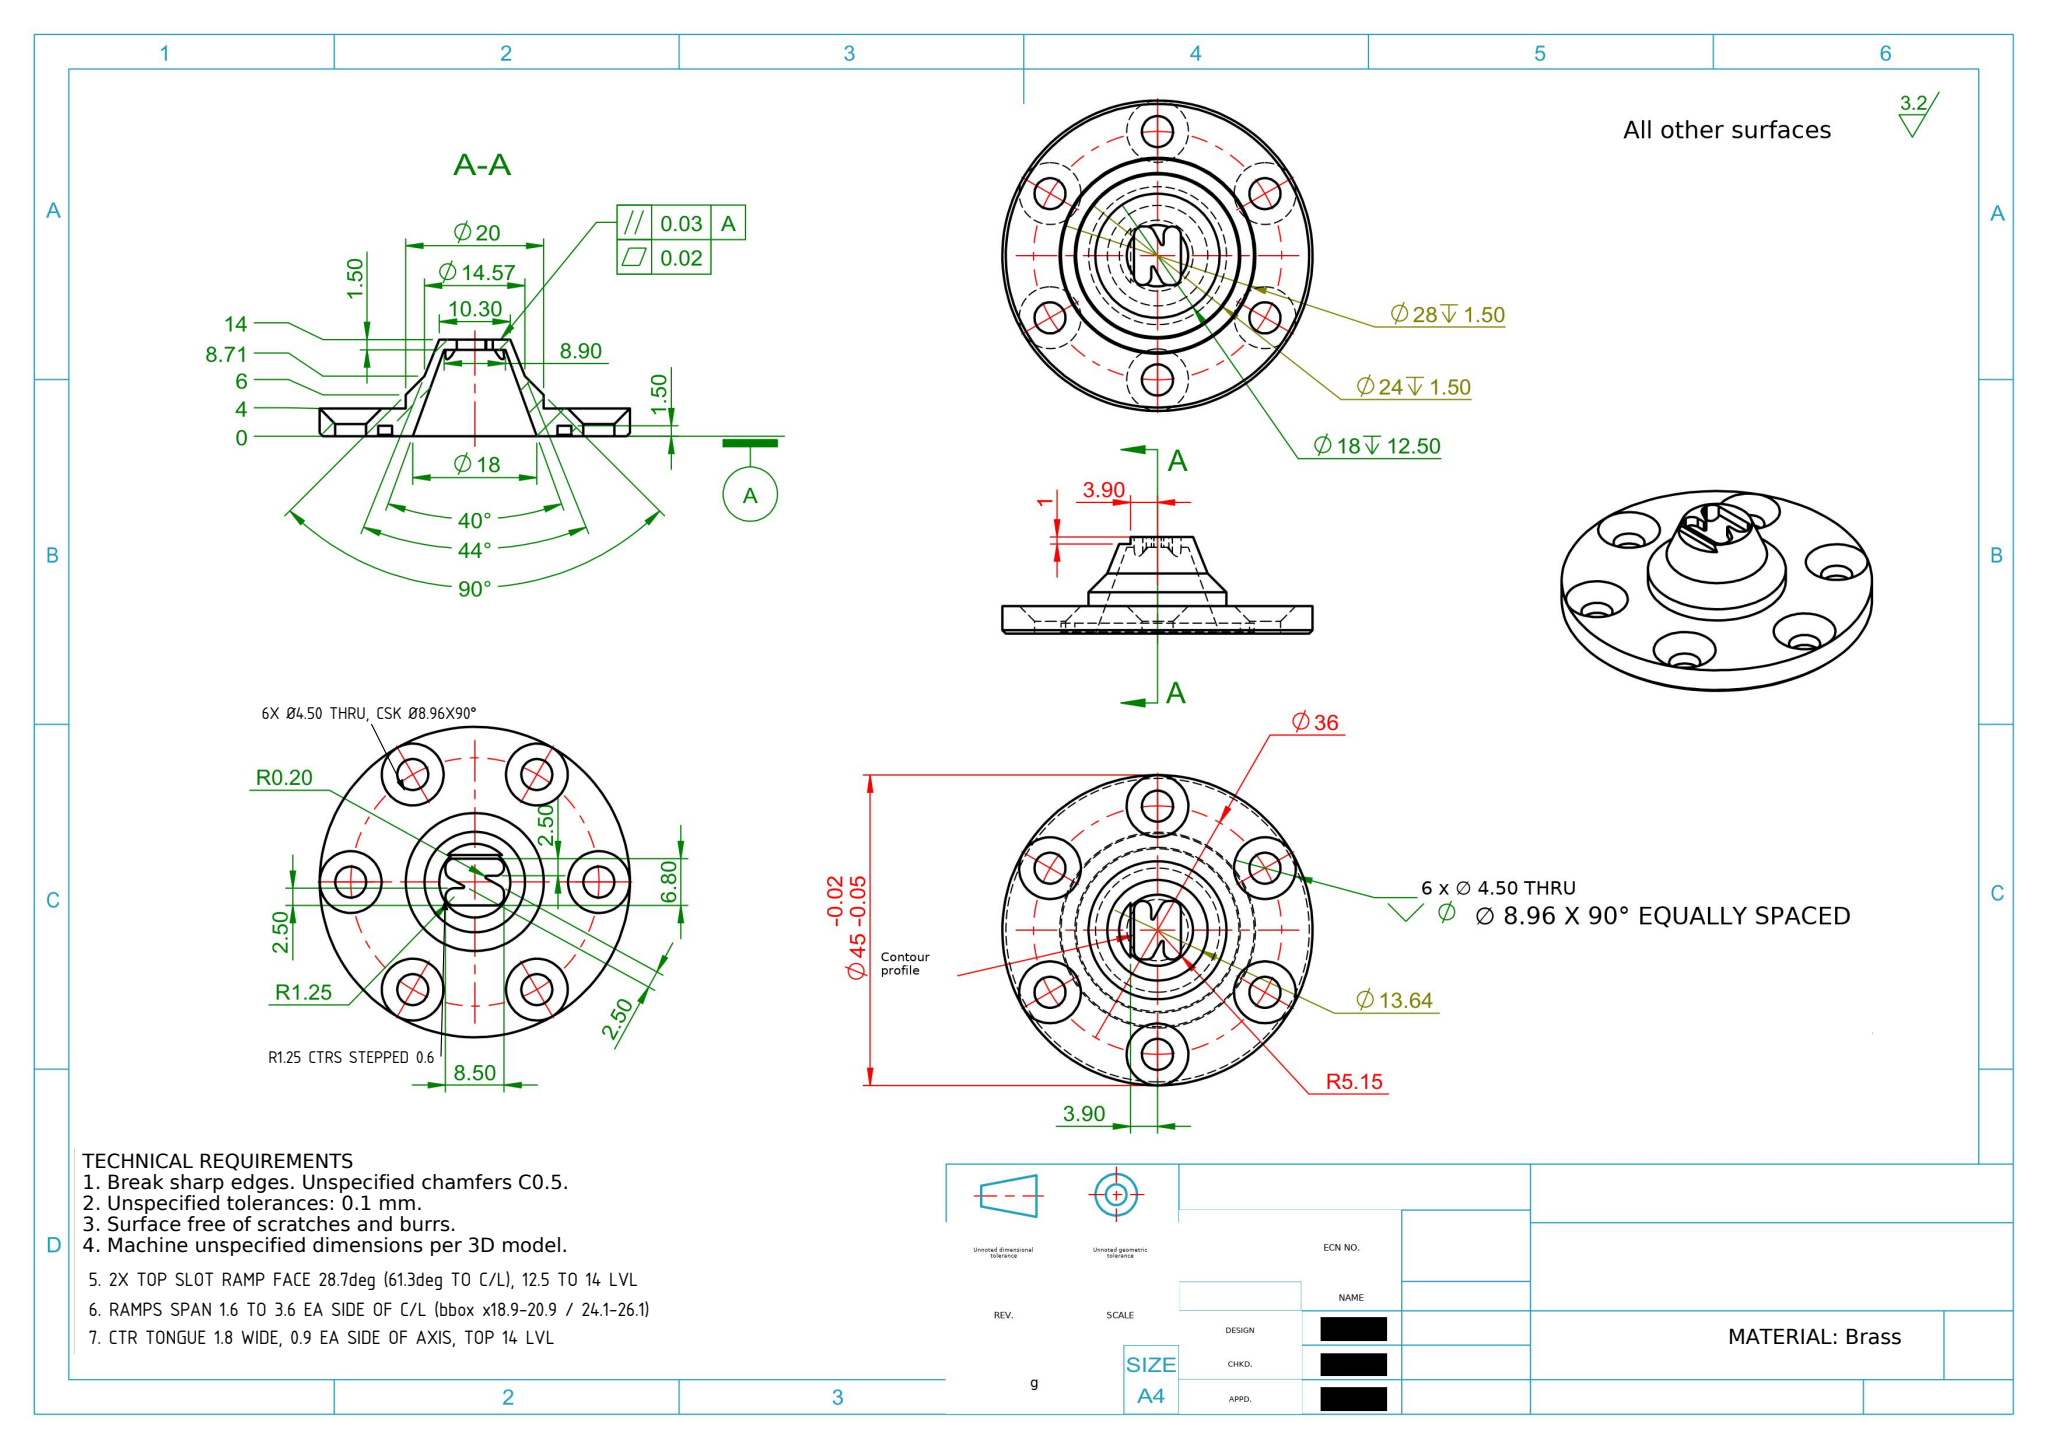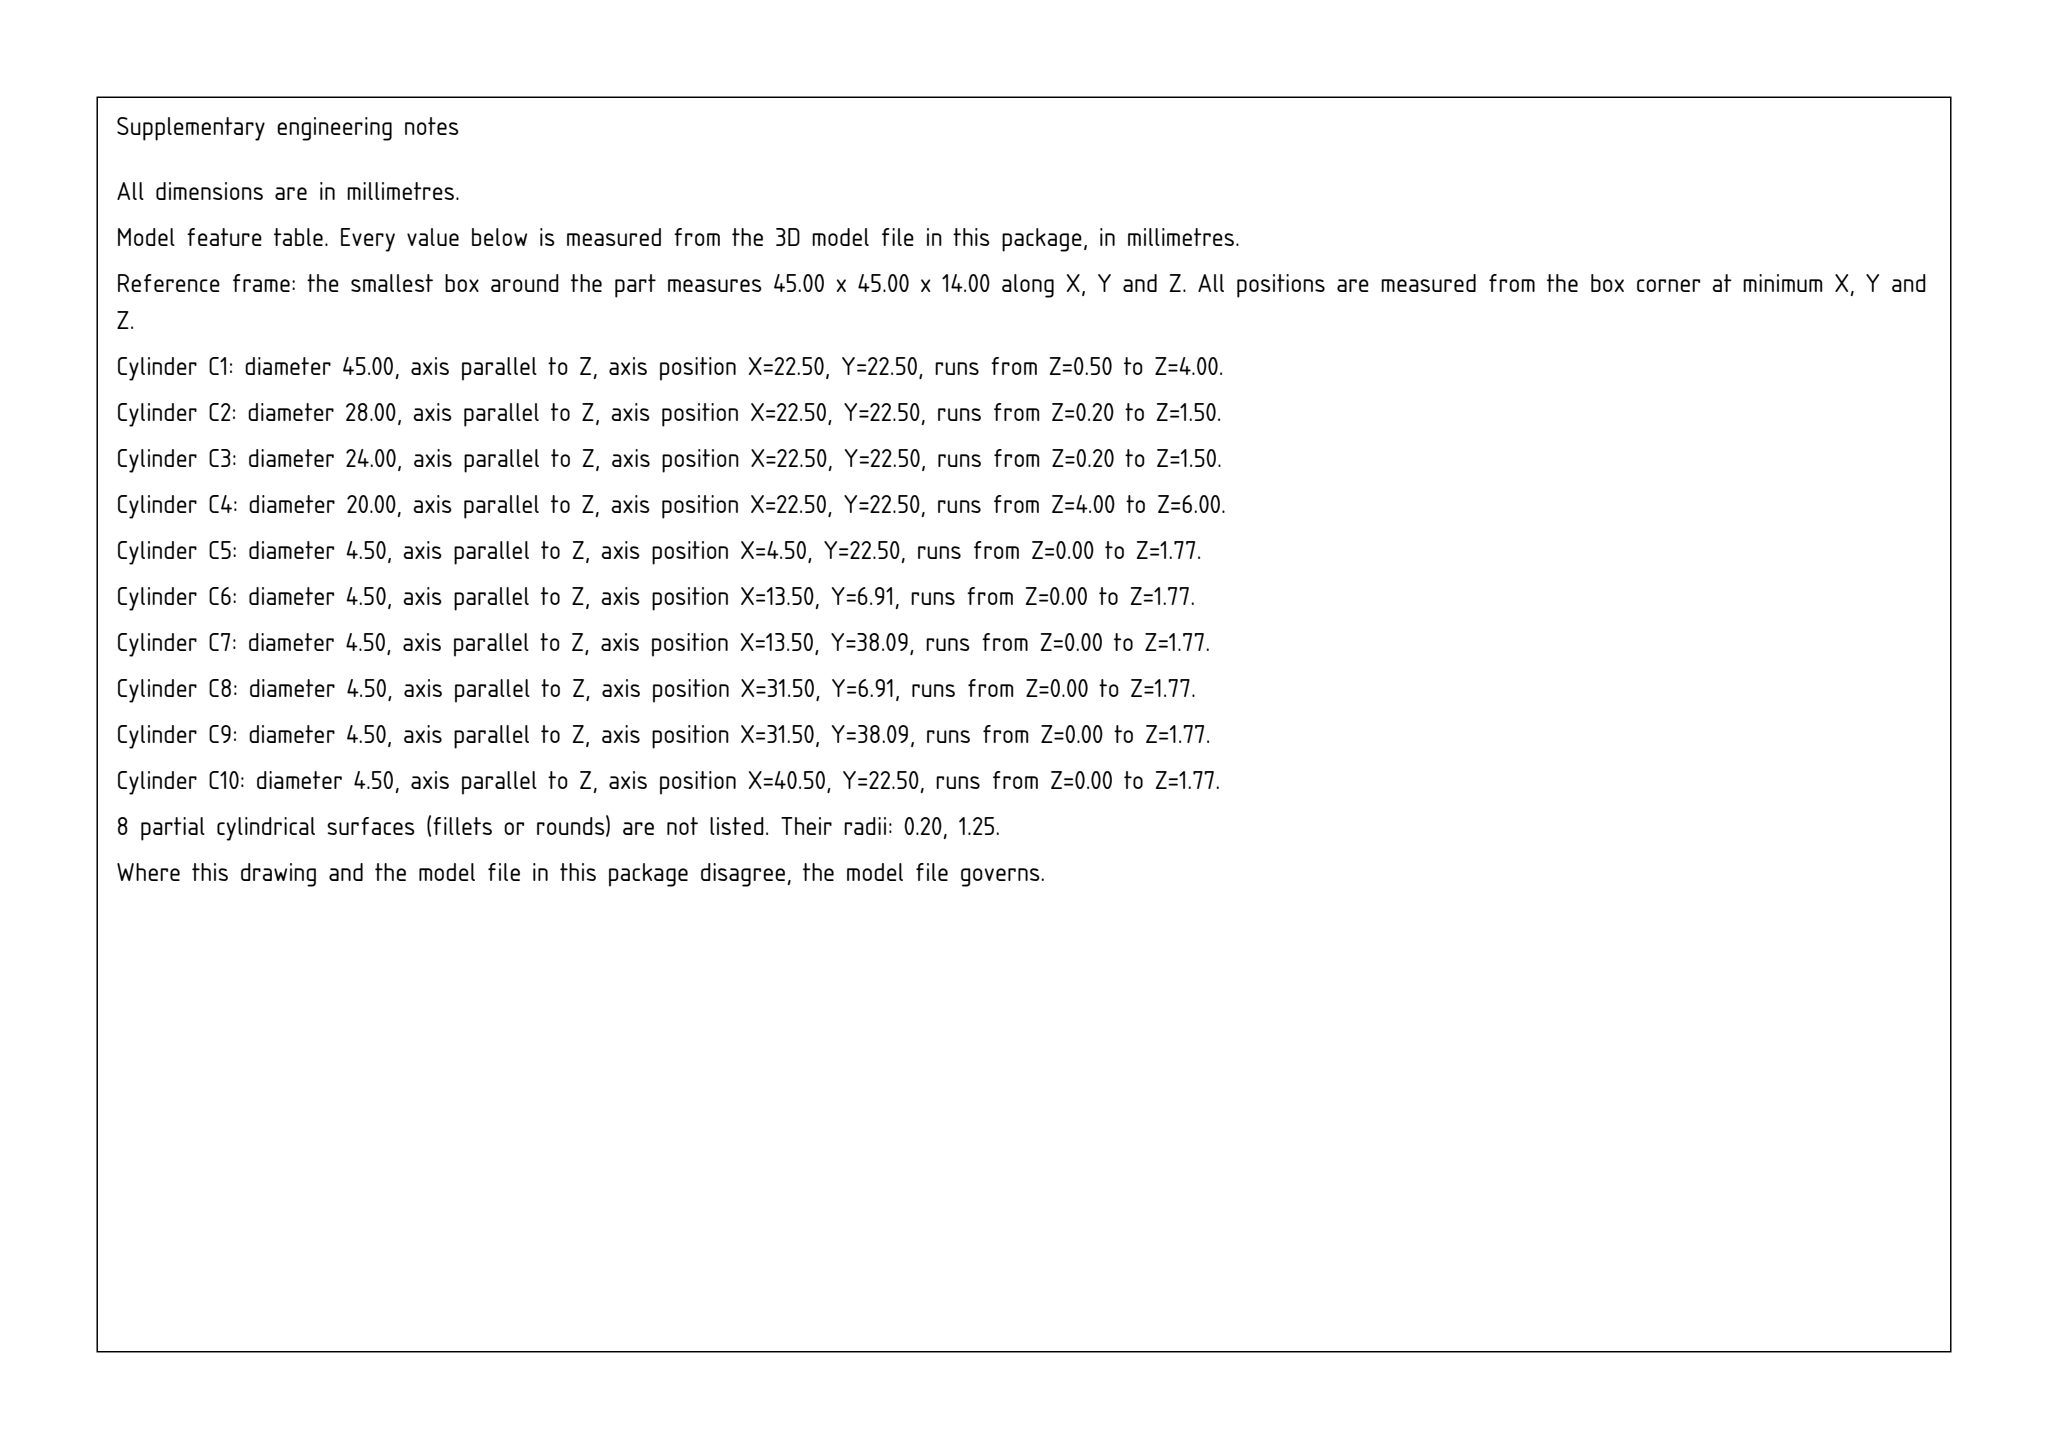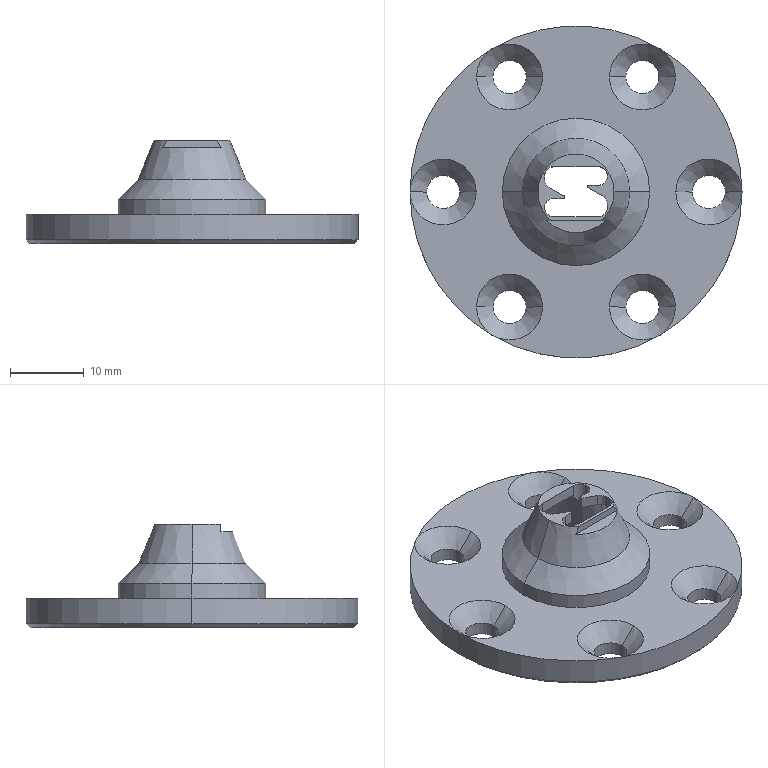Part | SolidWorks | mm | material Brass | 1 solid | 74 faces | box 45 x 45 x 14 mm | volume 5425 mm3 | cylinder 31 | cone 24 | plane 19 | commonest cylinder face diameters 4.5 x12 2.5 x8 0.4 x3 24 x2 28 x2 20 x2 45 x2
Drawing notes:
2X TOP SLOT RAMP FACE 28.7deg (61.3deg TO C/L), 12.5 TO 14 LVL | from the solid: inclined_planes angle_to_xyz [61.3,28.7,90.0], z 12.5->14.0, rise 1.5
RAMPS SPAN 1.6 TO 3.6 EA SIDE OF C/L (bbox x18.9-20.9 / 24.1-26.1) | from the solid: inclined bbox_from x=18.9 & 24.1, size x=2.0; part axis x=22.5
CTR TONGUE 1.8 WIDE, 0.9 EA SIDE OF AXIS, TOP 14 LVL | from the solid: planes y=21.6 & y=23.4 (axis y=22.5), z 12.5-14.0
R1.25 SLOT END ARC CTRS STEPPED 0.6 ACROSS SLOT | from the solid: arc dia 2.5 ctrs y=24.1 vs 24.7 at x=19.5; y=20.9 vs 20.4 at x=25.5
6X Ø4.50 THRU, CSK Ø8.96 X 90deg, EQ SP ON Ø36 B.C. | from the solid: 6 bores dia 4.5 thru, cones 90deg ref_dia 8.96; hole ctrs R18 from (22.5,22.5)